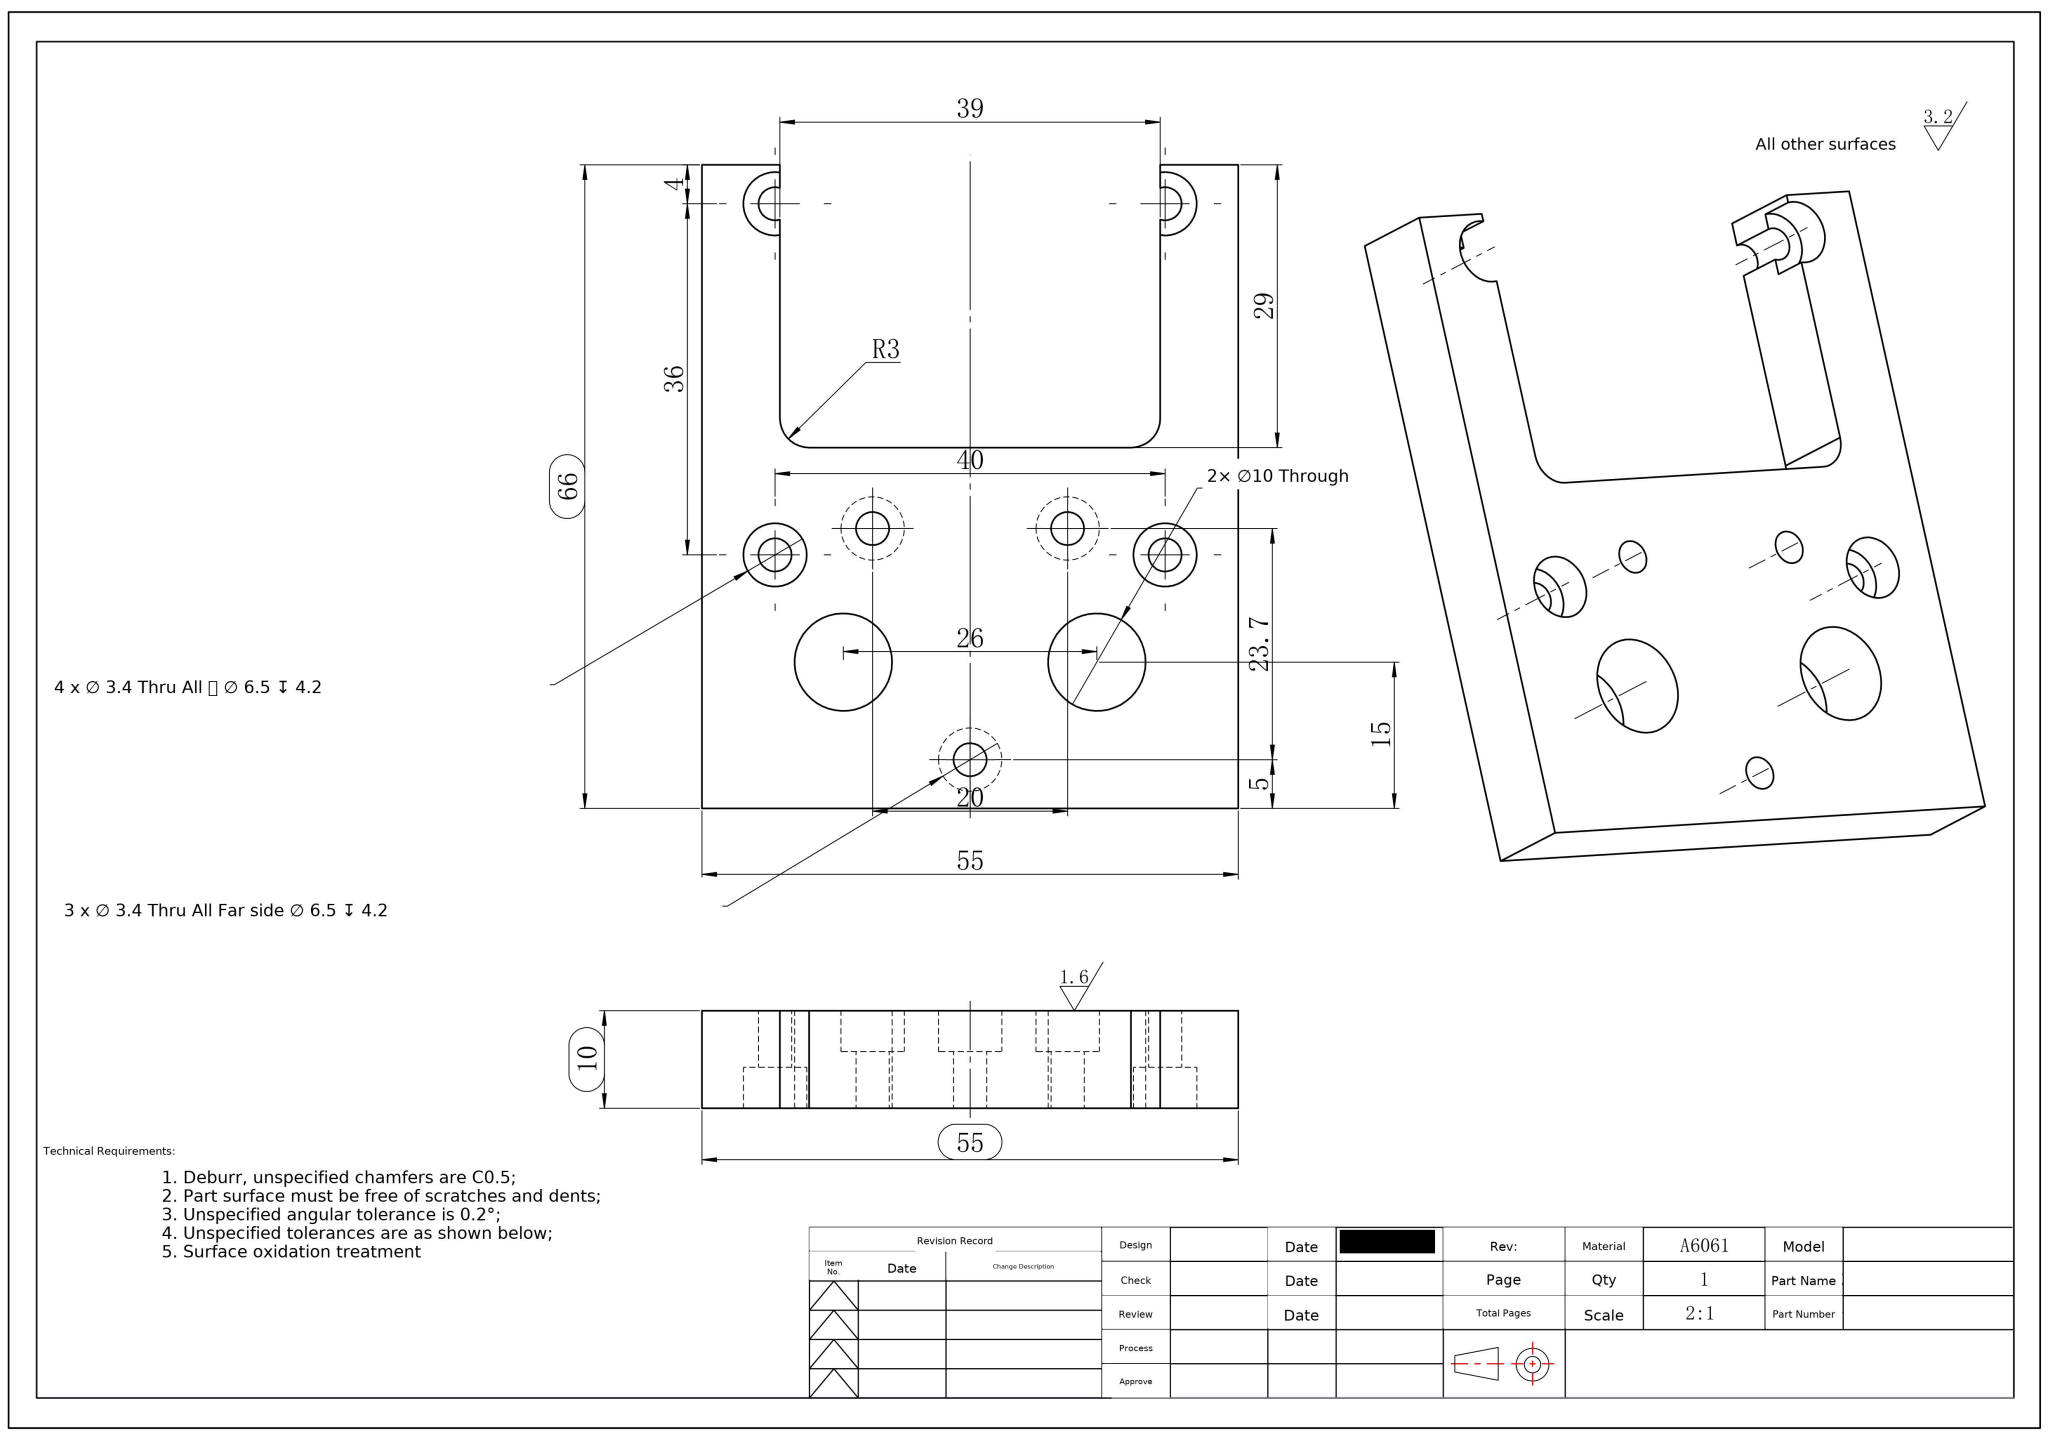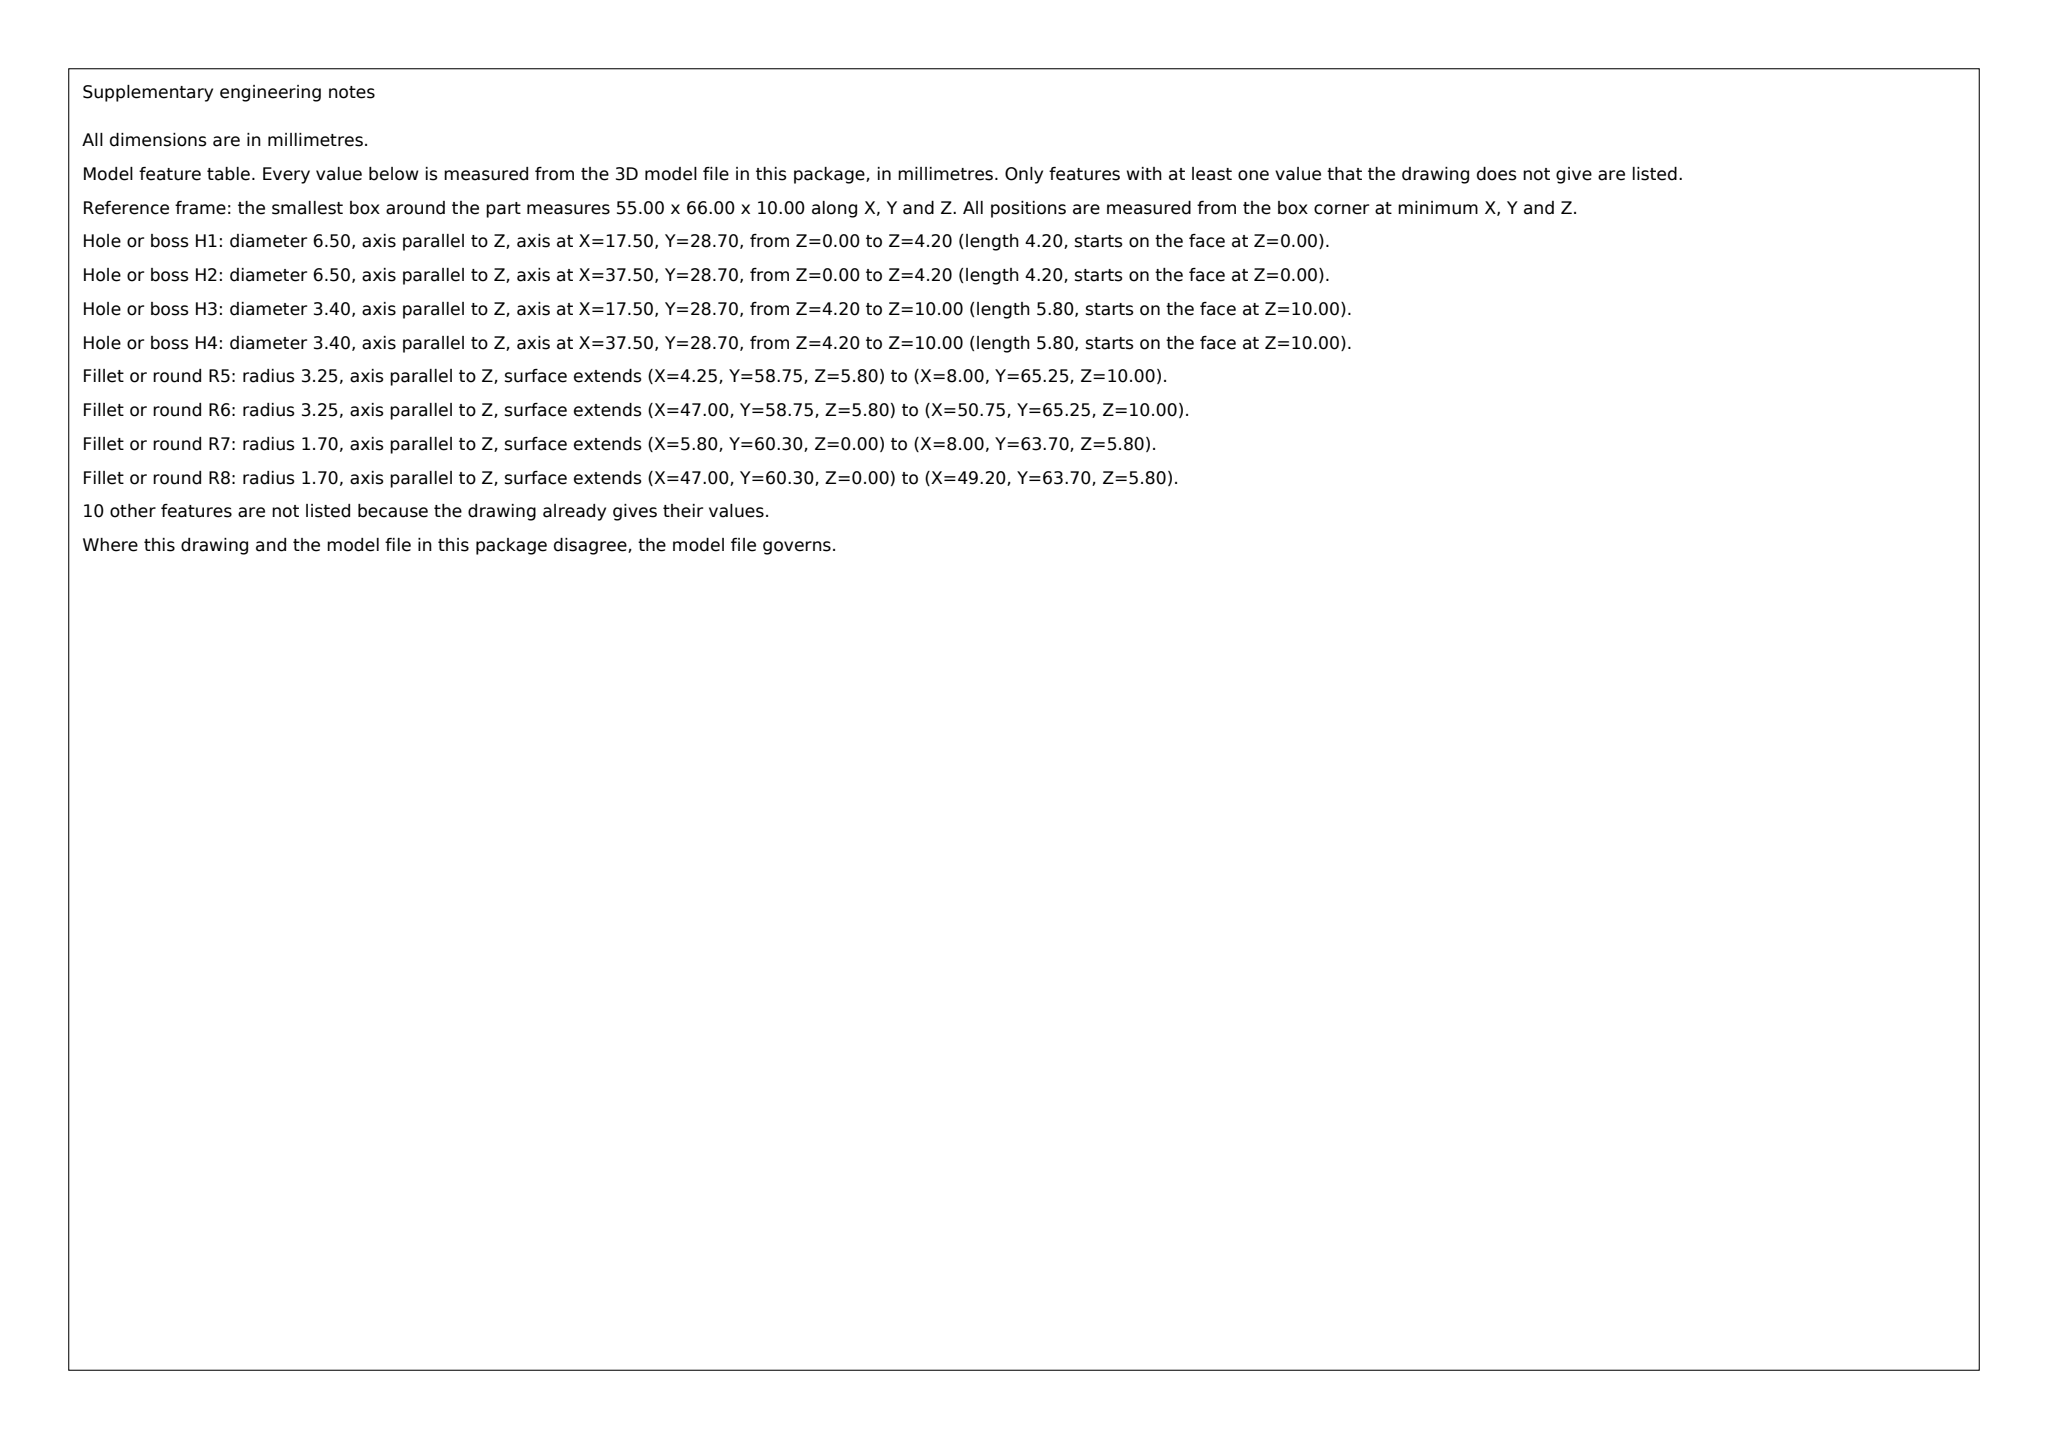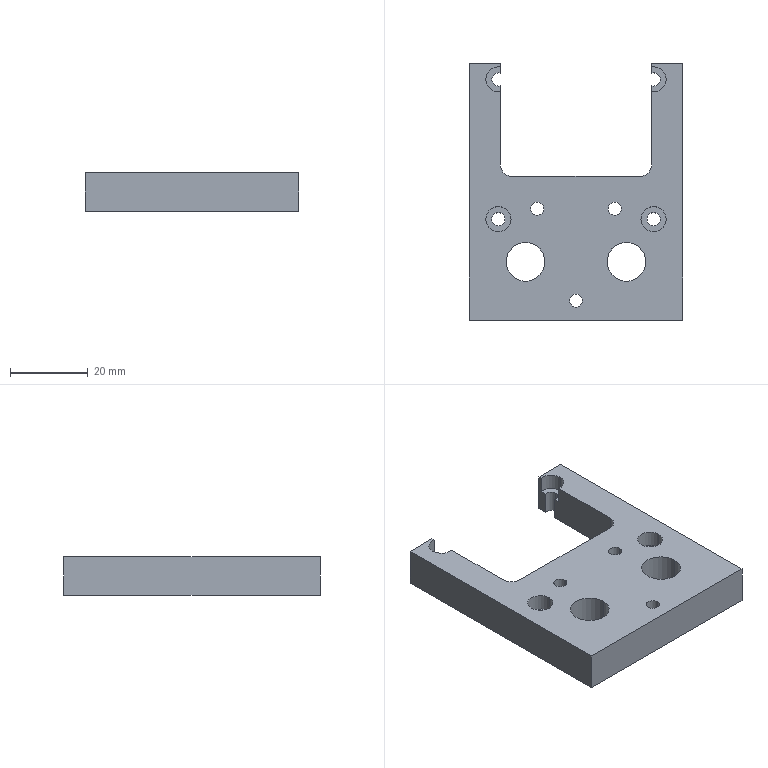Part | SolidWorks | mm | material A6061 | 1 solid | 51 faces | box 55 x 66 x 10 mm | volume 22259 mm3 | cylinder 32 | plane 19 | commonest cylinder face diameters 6.5 x13 3.4 x13 10 x4 6 x2
build123d program:
from build123d import *

# Parameters (mm, degrees)
SKETCH1_W                                       = 55
SKETCH1_H                                       = 66
BOSS_EXTRUDE1_DEPTH                             = 10
M3_HEX_SOCKET_HEAD_CAP_SCREW_CBORE2_D           = 3.4
M3_HEX_SOCKET_HEAD_CAP_SCREW_CBORE2_CBORE_D     = 6.5
M3_HEX_SOCKET_HEAD_CAP_SCREW_CBORE2_CBORE_DEPTH = 4.2
M3_HEX_SOCKET_HEAD_CAP_SCREW_CBORE3_D           = 3.4
M3_HEX_SOCKET_HEAD_CAP_SCREW_CBORE3_CBORE_D     = 6.5
M3_HEX_SOCKET_HEAD_CAP_SCREW_CBORE3_CBORE_DEPTH = 4.2
SKETCH8_W                                       = 39
SKETCH8_H                                       = 29
CUT_EXTRUDE1_DEPTH                              = 10
FILLET1_R                                       = 3
SKETCH9_R                                       = 5
CUT_EXTRUDE2_DEPTH                              = 45.105


with BuildPart() as part:
    # Sketch1 → Boss-Extrude1 (new body)
    with BuildSketch(Plane.XY):
        Rectangle(SKETCH1_W, SKETCH1_H)
    extrude(amount=BOSS_EXTRUDE1_DEPTH)

    # M3 Hex Socket Head Cap Screw CBORE2 (through all)
    with Locations(Plane.XY.offset(10)):
        with Locations((-20, 29), (-20, -7), (20, -7), (20, 29)):
            CounterBoreHole(M3_HEX_SOCKET_HEAD_CAP_SCREW_CBORE2_D / 2, M3_HEX_SOCKET_HEAD_CAP_SCREW_CBORE2_CBORE_D / 2, M3_HEX_SOCKET_HEAD_CAP_SCREW_CBORE2_CBORE_DEPTH)

    # M3 Hex Socket Head Cap Screw CBORE3 (through all)
    with Locations(Plane(origin=(0, 0, 0), x_dir=(-1, 0, 0), z_dir=(0, 0, -1))):
        with Locations((-10, -4.3), (0, -28), (10, -4.3)):
            CounterBoreHole(M3_HEX_SOCKET_HEAD_CAP_SCREW_CBORE3_D / 2, M3_HEX_SOCKET_HEAD_CAP_SCREW_CBORE3_CBORE_D / 2, M3_HEX_SOCKET_HEAD_CAP_SCREW_CBORE3_CBORE_DEPTH)

    # Sketch8 → Cut-Extrude1 (cut)
    with BuildSketch(Plane.XY.offset(10)):
        with Locations((0, 18.5)):
            Rectangle(SKETCH8_W, SKETCH8_H)
    extrude(amount=-CUT_EXTRUDE1_DEPTH, mode=Mode.SUBTRACT)

    # Fillet1
    fillet1_edges = [part.edges().sort_by_distance(p)[0] for p in [
        (-19.5, 4, 5),
        (19.5, 4, 5),
    ]]
    fillet(fillet1_edges, radius=FILLET1_R)

    # Sketch9 → Cut-Extrude2 (cut, through all)
    with BuildSketch(Plane.XY.offset(10)):
        with Locations((-13, -18)):
            Circle(SKETCH9_R)
        with Locations((13, -18)):
            Circle(SKETCH9_R)
    extrude(amount=-CUT_EXTRUDE2_DEPTH, mode=Mode.SUBTRACT)


solid = part.part